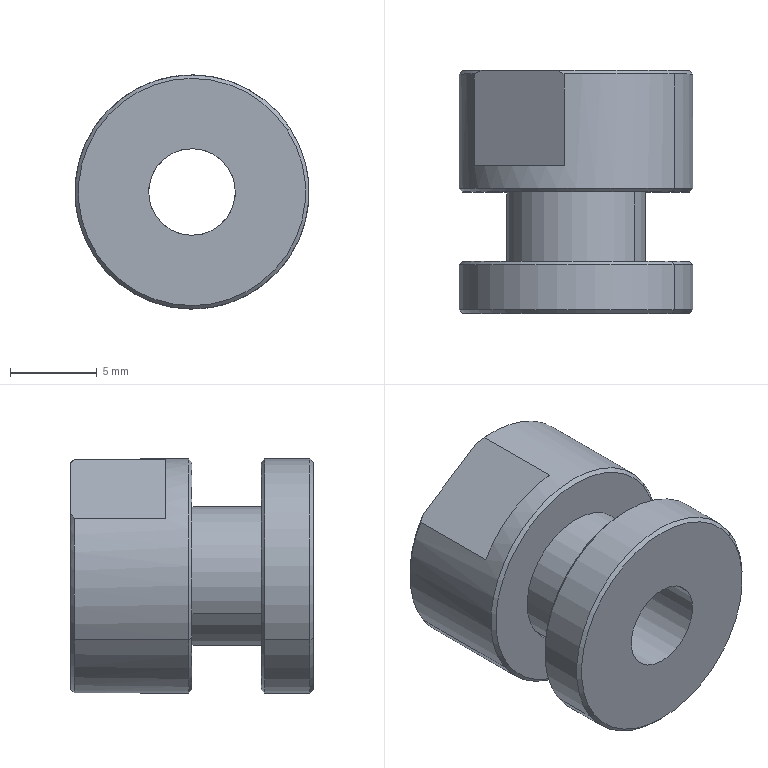Component | SolidWorks | WHC61-M5-0.8-L4.stp-1 | 1 solid | 25 faces | box 13.5 x 14 x 13.5 mm | volume 1320 mm3 | cone 9 | cylinder 8 | plane 8 | commonest cylinder face diameters 13.5 x4 5 x2 8 x2 | material AISI 304
STEP:
#1=COLOUR_RGB('',0.7922,0.8196,0.9333);
#2=FILL_AREA_STYLE_COLOUR('',#1);
#3=FILL_AREA_STYLE('',(#2));
#4=SURFACE_STYLE_FILL_AREA(#3);
#5=SURFACE_SIDE_STYLE('',(#4));
#6=SURFACE_STYLE_USAGE(.BOTH.,#5);
#7=PRESENTATION_STYLE_ASSIGNMENT((#6));
#8=CARTESIAN_POINT('',(0.08246,-2.402,0.05374));
#9=VERTEX_POINT('',#8);
#10=CARTESIAN_POINT('',(-0.08246,-2.402,-0.05374));
#11=VERTEX_POINT('',#10);
#12=CARTESIAN_POINT('',(0.,-2.402,0.));
#13=DIRECTION('',(0.,-1.,-0.));
#14=DIRECTION('',(-0.8378,0.,-0.546));
#15=AXIS2_PLACEMENT_3D('',#12,#13,#14);
#16=CIRCLE('',#15,0.09843);
#17=EDGE_CURVE('',#9,#11,#16,.T.);
#18=ORIENTED_EDGE('',*,*,#17,.F.);
#19=CARTESIAN_POINT('',(0.08246,-2.953,0.05374));
#20=VERTEX_POINT('',#19);
#21=CARTESIAN_POINT('',(0.08246,-2.402,0.05374));
#22=DIRECTION('',(0.,-1.,-0.));
#23=VECTOR('',#22,39.37);
#24=LINE('',#21,#23);
#25=EDGE_CURVE('',#9,#20,#24,.T.);
#26=ORIENTED_EDGE('',*,*,#25,.T.);
#27=CARTESIAN_POINT('',(-0.08246,-2.953,-0.05374));
#28=VERTEX_POINT('',#27);
#29=CARTESIAN_POINT('',(0.08246,-2.953,0.05374));
#30=CARTESIAN_POINT('',(0.07542,-2.953,0.06454));
#31=CARTESIAN_POINT('',(0.06624,-2.953,0.07393));
#32=CARTESIAN_POINT('',(0.04498,-2.953,0.08849));
#33=CARTESIAN_POINT('',(0.03291,-2.953,0.09365));
#34=CARTESIAN_POINT('',(0.007696,-2.953,0.09897));
#35=CARTESIAN_POINT('',(-0.005434,-2.953,0.09912));
#36=CARTESIAN_POINT('',(-0.03076,-2.953,0.09438));
#37=CARTESIAN_POINT('',(-0.04295,-2.953,0.08949));
#38=CARTESIAN_POINT('',(-0.06454,-2.953,0.07542));
#39=CARTESIAN_POINT('',(-0.07393,-2.953,0.06624));
#40=CARTESIAN_POINT('',(-0.08849,-2.953,0.04498));
#41=CARTESIAN_POINT('',(-0.09365,-2.953,0.03291));
#42=CARTESIAN_POINT('',(-0.09897,-2.953,0.007696));
#43=CARTESIAN_POINT('',(-0.09912,-2.953,-0.005434));
#44=CARTESIAN_POINT('',(-0.09438,-2.953,-0.03076));
#45=CARTESIAN_POINT('',(-0.08949,-2.953,-0.04295));
#46=CARTESIAN_POINT('',(-0.08246,-2.953,-0.05374));
#47=B_SPLINE_CURVE_WITH_KNOTS('',3,(#29,#30,#31,#32,#33,#34,#35,#36,#37,#38,#39,#40,#41,#42,#43,#44,#45,#46),.UNSPECIFIED.,.F.,.F.,(4,2,2,2,2,2,2,2,4),(0.5,0.5625,0.625,0.6875,0.75,0.8125,0.875,0.9375,1.),.UNSPECIFIED.);
#48=EDGE_CURVE('',#20,#28,#47,.T.);
#49=ORIENTED_EDGE('',*,*,#48,.T.);
#50=CARTESIAN_POINT('',(-0.08246,-2.402,-0.05374));
#51=DIRECTION('',(0.,-1.,-0.));
#52=VECTOR('',#51,39.37);
#53=LINE('',#50,#52);
#54=EDGE_CURVE('',#11,#28,#53,.T.);
#55=ORIENTED_EDGE('',*,*,#54,.F.);
#56=EDGE_LOOP('',(#18,#26,#49,#55));
#57=FACE_OUTER_BOUND('',#56,.T.);
#58=CARTESIAN_POINT('',(0.,-2.402,0.));
#59=DIRECTION('',(0.,-1.,-0.));
#60=DIRECTION('',(-0.8378,0.,-0.546));
#61=AXIS2_PLACEMENT_3D('',#58,#59,#60);
#62=CYLINDRICAL_SURFACE('',#61,0.09843);
#63=ADVANCED_FACE('',(#57),#62,.F.);
#64=CARTESIAN_POINT('',(-0.1319,-2.677,-0.08599));
#65=VERTEX_POINT('',#64);
#66=CARTESIAN_POINT('',(0.1319,-2.677,0.08599));
#67=VERTEX_POINT('',#66);
#68=CARTESIAN_POINT('',(0.,-2.677,0.));
#69=DIRECTION('',(-0.,1.,0.));
#70=DIRECTION('',(0.8378,0.,0.546));
#71=AXIS2_PLACEMENT_3D('',#68,#69,#70);
#72=CIRCLE('',#71,0.1575);
#73=EDGE_CURVE('',#65,#67,#72,.T.);
#74=ORIENTED_EDGE('',*,*,#73,.F.);
#75=CARTESIAN_POINT('',(-0.1319,-2.835,-0.08599));
#76=VERTEX_POINT('',#75);
#77=CARTESIAN_POINT('',(-0.1319,-0.9843,-0.08599));
#78=DIRECTION('',(0.,-1.,-0.));
#79=VECTOR('',#78,39.37);
#80=LINE('',#77,#79);
#81=EDGE_CURVE('',#65,#76,#80,.T.);
#82=ORIENTED_EDGE('',*,*,#81,.T.);
#83=CARTESIAN_POINT('',(0.1319,-2.835,0.08599));
#84=VERTEX_POINT('',#83);
#85=CARTESIAN_POINT('',(0.,-2.835,0.));
#86=DIRECTION('',(-0.,1.,0.));
#87=DIRECTION('',(0.8378,0.,0.546));
#88=AXIS2_PLACEMENT_3D('',#85,#86,#87);
#89=CIRCLE('',#88,0.1575);
#90=EDGE_CURVE('',#76,#84,#89,.T.);
#91=ORIENTED_EDGE('',*,*,#90,.T.);
#92=CARTESIAN_POINT('',(0.1319,-0.9843,0.08599));
#93=DIRECTION('',(0.,-1.,-0.));
#94=VECTOR('',#93,39.37);
#95=LINE('',#92,#94);
#96=EDGE_CURVE('',#67,#84,#95,.T.);
#97=ORIENTED_EDGE('',*,*,#96,.F.);
#98=EDGE_LOOP('',(#74,#82,#91,#97));
#99=FACE_OUTER_BOUND('',#98,.T.);
#100=CARTESIAN_POINT('',(-0.,-0.9843,0.));
#101=DIRECTION('',(0.,-1.,-0.));
#102=DIRECTION('',(0.8378,0.,0.546));
#103=AXIS2_PLACEMENT_3D('',#100,#101,#102);
#104=CYLINDRICAL_SURFACE('',#103,0.1575);
#105=ADVANCED_FACE('',(#99),#104,.T.);
#106=CARTESIAN_POINT('',(0.216,-2.835,0.1408));
#107=VERTEX_POINT('',#106);
#108=CARTESIAN_POINT('',(-0.216,-2.835,-0.1408));
#109=VERTEX_POINT('',#108);
#110=CARTESIAN_POINT('',(0.,-2.835,0.));
#111=DIRECTION('',(-0.,1.,0.));
#112=DIRECTION('',(0.8378,0.,0.546));
#113=AXIS2_PLACEMENT_3D('',#110,#111,#112);
#114=CIRCLE('',#113,0.2579);
#115=EDGE_CURVE('',#107,#109,#114,.T.);
#116=ORIENTED_EDGE('',*,*,#115,.F.);
#117=CARTESIAN_POINT('',(0.2226,-2.843,0.1451));
#118=VERTEX_POINT('',#117);
#119=CARTESIAN_POINT('',(0.2226,-2.843,0.1451));
#120=DIRECTION('',(0.5924,-0.7071,0.3861));
#121=VECTOR('',#120,39.37);
#122=LINE('',#119,#121);
#123=EDGE_CURVE('',#107,#118,#122,.T.);
#124=ORIENTED_EDGE('',*,*,#123,.T.);
#125=CARTESIAN_POINT('',(-0.2226,-2.843,-0.1451));
#126=VERTEX_POINT('',#125);
#127=CARTESIAN_POINT('',(0.,-2.843,0.));
#128=DIRECTION('',(-0.,1.,0.));
#129=DIRECTION('',(0.8378,0.,0.546));
#130=AXIS2_PLACEMENT_3D('',#127,#128,#129);
#131=CIRCLE('',#130,0.2657);
#132=EDGE_CURVE('',#118,#126,#131,.T.);
#133=ORIENTED_EDGE('',*,*,#132,.T.);
#134=CARTESIAN_POINT('',(-0.2226,-2.843,-0.1451));
#135=DIRECTION('',(-0.5924,-0.7071,-0.3861));
#136=VECTOR('',#135,39.37);
#137=LINE('',#134,#136);
#138=EDGE_CURVE('',#109,#126,#137,.T.);
#139=ORIENTED_EDGE('',*,*,#138,.F.);
#140=EDGE_LOOP('',(#116,#124,#133,#139));
#141=FACE_OUTER_BOUND('',#140,.T.);
#142=CARTESIAN_POINT('',(0.,-2.843,0.));
#143=DIRECTION('',(0.,-1.,-0.));
#144=DIRECTION('',(-0.8378,0.,-0.546));
#145=AXIS2_PLACEMENT_3D('',#142,#143,#144);
#146=CONICAL_SURFACE('',#145,0.2657,0.7854);
#147=ADVANCED_FACE('',(#141),#146,.T.);
#148=CARTESIAN_POINT('',(0.,-2.843,0.));
#149=DIRECTION('',(-0.,1.,0.));
#150=DIRECTION('',(0.8378,0.,0.546));
#151=AXIS2_PLACEMENT_3D('',#148,#149,#150);
#152=CIRCLE('',#151,0.2657);
#153=EDGE_CURVE('',#126,#118,#152,.T.);
#154=ORIENTED_EDGE('',*,*,#153,.F.);
#155=CARTESIAN_POINT('',(-0.2226,-2.945,-0.1451));
#156=VERTEX_POINT('',#155);
#157=CARTESIAN_POINT('',(-0.2226,-0.9843,-0.1451));
#158=DIRECTION('',(0.,-1.,-0.));
#159=VECTOR('',#158,39.37);
#160=LINE('',#157,#159);
#161=EDGE_CURVE('',#126,#156,#160,.T.);
#162=ORIENTED_EDGE('',*,*,#161,.T.);
#163=CARTESIAN_POINT('',(0.2226,-2.945,0.1451));
#164=VERTEX_POINT('',#163);
#165=CARTESIAN_POINT('',(0.,-2.945,0.));
#166=DIRECTION('',(-0.,1.,0.));
#167=DIRECTION('',(0.8378,0.,0.546));
#168=AXIS2_PLACEMENT_3D('',#165,#166,#167);
#169=CIRCLE('',#168,0.2657);
#170=EDGE_CURVE('',#156,#164,#169,.T.);
#171=ORIENTED_EDGE('',*,*,#170,.T.);
#172=CARTESIAN_POINT('',(0.2226,-0.9843,0.1451));
#173=DIRECTION('',(0.,-1.,-0.));
#174=VECTOR('',#173,39.37);
#175=LINE('',#172,#174);
#176=EDGE_CURVE('',#118,#164,#175,.T.);
#177=ORIENTED_EDGE('',*,*,#176,.F.);
#178=EDGE_LOOP('',(#154,#162,#171,#177));
#179=FACE_OUTER_BOUND('',#178,.T.);
#180=CARTESIAN_POINT('',(-0.,-0.9843,0.));
#181=DIRECTION('',(0.,-1.,-0.));
#182=DIRECTION('',(0.8378,0.,0.546));
#183=AXIS2_PLACEMENT_3D('',#180,#181,#182);
#184=CYLINDRICAL_SURFACE('',#183,0.2657);
#185=ADVANCED_FACE('',(#179),#184,.T.);
#186=CARTESIAN_POINT('',(0.216,-2.953,0.1408));
#187=VERTEX_POINT('',#186);
#188=CARTESIAN_POINT('',(-0.216,-2.953,-0.1408));
#189=VERTEX_POINT('',#188);
#190=CARTESIAN_POINT('',(0.,-2.953,0.));
#191=DIRECTION('',(-0.,1.,0.));
#192=DIRECTION('',(0.8378,0.,0.546));
#193=AXIS2_PLACEMENT_3D('',#190,#191,#192);
#194=CIRCLE('',#193,0.2579);
#195=EDGE_CURVE('',#187,#189,#194,.T.);
#196=ORIENTED_EDGE('',*,*,#195,.T.);
#197=CARTESIAN_POINT('',(-0.216,-2.953,-0.1408));
#198=DIRECTION('',(-0.5924,0.7071,-0.3861));
#199=VECTOR('',#198,39.37);
#200=LINE('',#197,#199);
#201=EDGE_CURVE('',#189,#156,#200,.T.);
#202=ORIENTED_EDGE('',*,*,#201,.T.);
#203=CARTESIAN_POINT('',(0.,-2.945,0.));
#204=DIRECTION('',(-0.,1.,0.));
#205=DIRECTION('',(0.8378,0.,0.546));
#206=AXIS2_PLACEMENT_3D('',#203,#204,#205);
#207=CIRCLE('',#206,0.2657);
#208=EDGE_CURVE('',#164,#156,#207,.T.);
#209=ORIENTED_EDGE('',*,*,#208,.F.);
#210=CARTESIAN_POINT('',(0.216,-2.953,0.1408));
#211=DIRECTION('',(0.5924,0.7071,0.3861));
#212=VECTOR('',#211,39.37);
#213=LINE('',#210,#212);
#214=EDGE_CURVE('',#187,#164,#213,.T.);
#215=ORIENTED_EDGE('',*,*,#214,.F.);
#216=EDGE_LOOP('',(#196,#202,#209,#215));
#217=FACE_OUTER_BOUND('',#216,.T.);
#218=CARTESIAN_POINT('',(0.,-2.953,0.));
#219=DIRECTION('',(-0.,1.,0.));
#220=DIRECTION('',(0.8378,0.,0.546));
#221=AXIS2_PLACEMENT_3D('',#218,#219,#220);
#222=CONICAL_SURFACE('',#221,0.2579,0.7854);
#223=ADVANCED_FACE('',(#217),#222,.T.);
#224=CARTESIAN_POINT('',(0.216,-2.677,0.1408));
#225=VERTEX_POINT('',#224);
#226=CARTESIAN_POINT('',(-0.216,-2.677,-0.1408));
#227=VERTEX_POINT('',#226);
#228=CARTESIAN_POINT('',(0.,-2.677,0.));
#229=DIRECTION('',(-0.,1.,0.));
#230=DIRECTION('',(0.8378,0.,0.546));
#231=AXIS2_PLACEMENT_3D('',#228,#229,#230);
#232=CIRCLE('',#231,0.2579);
#233=EDGE_CURVE('',#225,#227,#232,.T.);
#234=ORIENTED_EDGE('',*,*,#233,.T.);
#235=CARTESIAN_POINT('',(-0.2226,-2.669,-0.1451));
#236=VERTEX_POINT('',#235);
#237=CARTESIAN_POINT('',(-0.216,-2.677,-0.1408));
#238=DIRECTION('',(-0.5924,0.7071,-0.3861));
#239=VECTOR('',#238,39.37);
#240=LINE('',#237,#239);
#241=EDGE_CURVE('',#227,#236,#240,.T.);
#242=ORIENTED_EDGE('',*,*,#241,.T.);
#243=CARTESIAN_POINT('',(0.2226,-2.669,0.1451));
#244=VERTEX_POINT('',#243);
#245=CARTESIAN_POINT('',(0.,-2.669,0.));
#246=DIRECTION('',(-0.,1.,0.));
#247=DIRECTION('',(0.8378,0.,0.546));
#248=AXIS2_PLACEMENT_3D('',#245,#246,#247);
#249=CIRCLE('',#248,0.2657);
#250=EDGE_CURVE('',#244,#236,#249,.T.);
#251=ORIENTED_EDGE('',*,*,#250,.F.);
#252=CARTESIAN_POINT('',(0.216,-2.677,0.1408));
#253=DIRECTION('',(0.5924,0.7071,0.3861));
#254=VECTOR('',#253,39.37);
#255=LINE('',#252,#254);
#256=EDGE_CURVE('',#225,#244,#255,.T.);
#257=ORIENTED_EDGE('',*,*,#256,.F.);
#258=EDGE_LOOP('',(#234,#242,#251,#257));
#259=FACE_OUTER_BOUND('',#258,.T.);
#260=CARTESIAN_POINT('',(0.,-2.677,0.));
#261=DIRECTION('',(-0.,1.,0.));
#262=DIRECTION('',(0.8378,0.,0.546));
#263=AXIS2_PLACEMENT_3D('',#260,#261,#262);
#264=CONICAL_SURFACE('',#263,0.2579,0.7854);
#265=ADVANCED_FACE('',(#259),#264,.T.);
#266=CARTESIAN_POINT('',(-0.216,-2.402,-0.1408));
#267=VERTEX_POINT('',#266);
#268=CARTESIAN_POINT('',(-0.2156,-2.402,0.1414));
#269=VERTEX_POINT('',#268);
#270=CARTESIAN_POINT('',(0.,-2.402,0.));
#271=DIRECTION('',(-0.,1.,0.));
#272=DIRECTION('',(0.8378,0.,0.546));
#273=AXIS2_PLACEMENT_3D('',#270,#271,#272);
#274=CIRCLE('',#273,0.2579);
#275=EDGE_CURVE('',#267,#269,#274,.T.);
#276=ORIENTED_EDGE('',*,*,#275,.F.);
#277=CARTESIAN_POINT('',(-0.2226,-2.409,-0.1451));
#278=VERTEX_POINT('',#277);
#279=CARTESIAN_POINT('',(-0.2226,-2.409,-0.1451));
#280=DIRECTION('',(-0.5924,-0.7071,-0.3861));
#281=VECTOR('',#280,39.37);
#282=LINE('',#279,#281);
#283=EDGE_CURVE('',#267,#278,#282,.T.);
#284=ORIENTED_EDGE('',*,*,#283,.T.);
#285=CARTESIAN_POINT('',(-0.231,-2.409,0.1314));
#286=VERTEX_POINT('',#285);
#287=CARTESIAN_POINT('',(0.,-2.409,0.));
#288=DIRECTION('',(-0.,1.,0.));
#289=DIRECTION('',(0.8378,0.,0.546));
#290=AXIS2_PLACEMENT_3D('',#287,#288,#289);
#291=CIRCLE('',#290,0.2657);
#292=EDGE_CURVE('',#278,#286,#291,.T.);
#293=ORIENTED_EDGE('',*,*,#292,.T.);
#294=CARTESIAN_POINT('',(-0.231,-2.409,0.1314));
#295=CARTESIAN_POINT('',(-0.2259,-2.407,0.1347));
#296=CARTESIAN_POINT('',(-0.2208,-2.404,0.138));
#297=CARTESIAN_POINT('',(-0.2156,-2.402,0.1414));
#298=B_SPLINE_CURVE_WITH_KNOTS('',3,(#294,#295,#296,#297),.UNSPECIFIED.,.F.,.F.,(4,4),(0.004377,0.00488),.UNSPECIFIED.);
#299=EDGE_CURVE('',#286,#269,#298,.T.);
#300=ORIENTED_EDGE('',*,*,#299,.T.);
#301=EDGE_LOOP('',(#276,#284,#293,#300));
#302=FACE_OUTER_BOUND('',#301,.T.);
#303=CARTESIAN_POINT('',(0.,-2.409,0.));
#304=DIRECTION('',(0.,-1.,-0.));
#305=DIRECTION('',(-0.8378,0.,-0.546));
#306=AXIS2_PLACEMENT_3D('',#303,#304,#305);
#307=CONICAL_SURFACE('',#306,0.2657,0.7854);
#308=ADVANCED_FACE('',(#302),#307,.T.);
#309=ORIENTED_EDGE('',*,*,#292,.F.);
#310=CARTESIAN_POINT('',(-0.2226,-0.9843,-0.1451));
#311=DIRECTION('',(0.,-1.,-0.));
#312=VECTOR('',#311,39.37);
#313=LINE('',#310,#312);
#314=EDGE_CURVE('',#278,#236,#313,.T.);
#315=ORIENTED_EDGE('',*,*,#314,.T.);
#316=CARTESIAN_POINT('',(0.,-2.669,0.));
#317=DIRECTION('',(-0.,1.,0.));
#318=DIRECTION('',(0.8378,0.,0.546));
#319=AXIS2_PLACEMENT_3D('',#316,#317,#318);
#320=CIRCLE('',#319,0.2657);
#321=EDGE_CURVE('',#236,#244,#320,.T.);
#322=ORIENTED_EDGE('',*,*,#321,.T.);
#323=CARTESIAN_POINT('',(0.2226,-2.409,0.1451));
#324=VERTEX_POINT('',#323);
#325=CARTESIAN_POINT('',(0.2226,-0.9843,0.1451));
#326=DIRECTION('',(0.,-1.,-0.));
#327=VECTOR('',#326,39.37);
#328=LINE('',#325,#327);
#329=EDGE_CURVE('',#324,#244,#328,.T.);
#330=ORIENTED_EDGE('',*,*,#329,.F.);
#331=CARTESIAN_POINT('',(-0.02699,-2.409,0.2644));
#332=VERTEX_POINT('',#331);
#333=CARTESIAN_POINT('',(0.,-2.409,0.));
#334=DIRECTION('',(-0.,1.,0.));
#335=DIRECTION('',(0.8378,0.,0.546));
#336=AXIS2_PLACEMENT_3D('',#333,#334,#335);
#337=CIRCLE('',#336,0.2657);
#338=EDGE_CURVE('',#332,#324,#337,.T.);
#339=ORIENTED_EDGE('',*,*,#338,.F.);
#340=CARTESIAN_POINT('',(-0.02699,-2.618,0.2644));
#341=VERTEX_POINT('',#340);
#342=CARTESIAN_POINT('',(-0.02699,-2.618,0.2644));
#343=DIRECTION('',(-0.,1.,0.));
#344=VECTOR('',#343,39.37);
#345=LINE('',#342,#344);
#346=EDGE_CURVE('',#341,#332,#345,.T.);
#347=ORIENTED_EDGE('',*,*,#346,.F.);
#348=CARTESIAN_POINT('',(-0.231,-2.618,0.1314));
#349=VERTEX_POINT('',#348);
#350=CARTESIAN_POINT('',(0.,-2.618,0.));
#351=DIRECTION('',(-0.,1.,0.));
#352=DIRECTION('',(0.546,0.,-0.8378));
#353=AXIS2_PLACEMENT_3D('',#350,#351,#352);
#354=CIRCLE('',#353,0.2657);
#355=EDGE_CURVE('',#349,#341,#354,.T.);
#356=ORIENTED_EDGE('',*,*,#355,.F.);
#357=CARTESIAN_POINT('',(-0.231,-2.618,0.1314));
#358=DIRECTION('',(-0.,1.,0.));
#359=VECTOR('',#358,39.37);
#360=LINE('',#357,#359);
#361=EDGE_CURVE('',#349,#286,#360,.T.);
#362=ORIENTED_EDGE('',*,*,#361,.T.);
#363=EDGE_LOOP('',(#309,#315,#322,#330,#339,#347,#356,#362));
#364=FACE_OUTER_BOUND('',#363,.T.);
#365=CARTESIAN_POINT('',(-0.,-0.9843,0.));
#366=DIRECTION('',(0.,-1.,-0.));
#367=DIRECTION('',(0.8378,0.,0.546));
#368=AXIS2_PLACEMENT_3D('',#365,#366,#367);
#369=CYLINDRICAL_SURFACE('',#368,0.2657);
#370=ADVANCED_FACE('',(#364),#369,.T.);
#371=ORIENTED_EDGE('',*,*,#195,.F.);
#372=CARTESIAN_POINT('',(0.,-2.953,0.));
#373=DIRECTION('',(-0.,1.,0.));
#374=DIRECTION('',(0.8378,0.,0.546));
#375=AXIS2_PLACEMENT_3D('',#372,#373,#374);
#376=CIRCLE('',#375,0.2579);
#377=EDGE_CURVE('',#189,#187,#376,.T.);
#378=ORIENTED_EDGE('',*,*,#377,.F.);
#379=EDGE_LOOP('',(#371,#378));
#380=FACE_OUTER_BOUND('',#379,.T.);
#381=CARTESIAN_POINT('',(-0.08246,-2.953,-0.05374));
#382=CARTESIAN_POINT('',(-0.07542,-2.953,-0.06454));
#383=CARTESIAN_POINT('',(-0.06624,-2.953,-0.07393));
#384=CARTESIAN_POINT('',(-0.04498,-2.953,-0.08849));
#385=CARTESIAN_POINT('',(-0.03291,-2.953,-0.09365));
#386=CARTESIAN_POINT('',(-0.007696,-2.953,-0.09897));
#387=CARTESIAN_POINT('',(0.005434,-2.953,-0.09912));
#388=CARTESIAN_POINT('',(0.03076,-2.953,-0.09438));
#389=CARTESIAN_POINT('',(0.04295,-2.953,-0.08949));
#390=CARTESIAN_POINT('',(0.06454,-2.953,-0.07542));
#391=CARTESIAN_POINT('',(0.07393,-2.953,-0.06624));
#392=CARTESIAN_POINT('',(0.08849,-2.953,-0.04498));
#393=CARTESIAN_POINT('',(0.09365,-2.953,-0.03291));
#394=CARTESIAN_POINT('',(0.09897,-2.953,-0.007696));
#395=CARTESIAN_POINT('',(0.09912,-2.953,0.005434));
#396=CARTESIAN_POINT('',(0.09438,-2.953,0.03076));
#397=CARTESIAN_POINT('',(0.08949,-2.953,0.04295));
#398=CARTESIAN_POINT('',(0.08246,-2.953,0.05374));
#399=B_SPLINE_CURVE_WITH_KNOTS('',3,(#381,#382,#383,#384,#385,#386,#387,#388,#389,#390,#391,#392,#393,#394,#395,#396,#397,#398),.UNSPECIFIED.,.F.,.F.,(4,2,2,2,2,2,2,2,4),(0.,0.0625,0.125,0.1875,0.25,0.3125,0.375,0.4375,0.5),.UNSPECIFIED.);
#400=EDGE_CURVE('',#28,#20,#399,.T.);
#401=ORIENTED_EDGE('',*,*,#400,.F.);
#402=ORIENTED_EDGE('',*,*,#48,.F.);
#403=EDGE_LOOP('',(#401,#402));
#404=FACE_BOUND('',#403,.T.);
#405=CARTESIAN_POINT('',(0.,-2.953,0.));
#406=DIRECTION('',(-0.,1.,0.));
#407=DIRECTION('',(-0.546,-0.,0.8378));
#408=AXIS2_PLACEMENT_3D('',#405,#406,#407);
#409=PLANE('',#408);
#410=ADVANCED_FACE('',(#380,#404),#409,.F.);
#411=ORIENTED_EDGE('',*,*,#361,.F.);
#412=CARTESIAN_POINT('',(-0.02699,-2.618,0.2644));
#413=DIRECTION('',(-0.8378,-0.,-0.546));
#414=VECTOR('',#413,39.37);
#415=LINE('',#412,#414);
#416=EDGE_CURVE('',#341,#349,#415,.T.);
#417=ORIENTED_EDGE('',*,*,#416,.F.);
#418=ORIENTED_EDGE('',*,*,#346,.T.);
#419=CARTESIAN_POINT('',(-0.04233,-2.402,0.2544));
#420=VERTEX_POINT('',#419);
#421=CARTESIAN_POINT('',(-0.04233,-2.402,0.2544));
#422=CARTESIAN_POINT('',(-0.03717,-2.404,0.2577));
#423=CARTESIAN_POINT('',(-0.03205,-2.407,0.2611));
#424=CARTESIAN_POINT('',(-0.02699,-2.409,0.2644));
#425=B_SPLINE_CURVE_WITH_KNOTS('',3,(#421,#422,#423,#424),.UNSPECIFIED.,.F.,.F.,(4,4),(0.01023,0.01072),.UNSPECIFIED.);
#426=EDGE_CURVE('',#420,#332,#425,.T.);
#427=ORIENTED_EDGE('',*,*,#426,.F.);
#428=CARTESIAN_POINT('',(-0.129,-2.402,0.1979));
#429=DIRECTION('',(0.8378,0.,0.546));
#430=VECTOR('',#429,39.37);
#431=LINE('',#428,#430);
#432=EDGE_CURVE('',#269,#420,#431,.T.);
#433=ORIENTED_EDGE('',*,*,#432,.F.);
#434=ORIENTED_EDGE('',*,*,#299,.F.);
#435=EDGE_LOOP('',(#411,#417,#418,#427,#433,#434));
#436=FACE_OUTER_BOUND('',#435,.T.);
#437=CARTESIAN_POINT('',(-0.02699,-2.618,0.2644));
#438=DIRECTION('',(0.546,0.,-0.8378));
#439=DIRECTION('',(-0.8378,-0.,-0.546));
#440=AXIS2_PLACEMENT_3D('',#437,#438,#439);
#441=PLANE('',#440);
#442=ADVANCED_FACE('',(#436),#441,.F.);
#443=ORIENTED_EDGE('',*,*,#416,.T.);
#444=ORIENTED_EDGE('',*,*,#355,.T.);
#445=EDGE_LOOP('',(#443,#444));
#446=FACE_OUTER_BOUND('',#445,.T.);
#447=CARTESIAN_POINT('',(0.,-2.618,0.));
#448=DIRECTION('',(-0.,1.,0.));
#449=DIRECTION('',(-0.546,-0.,0.8378));
#450=AXIS2_PLACEMENT_3D('',#447,#448,#449);
#451=PLANE('',#450);
#452=ADVANCED_FACE('',(#446),#451,.T.);
#453=ORIENTED_EDGE('',*,*,#314,.F.);
#454=CARTESIAN_POINT('',(0.02699,-2.409,-0.2644));
#455=VERTEX_POINT('',#454);
#456=CARTESIAN_POINT('',(0.,-2.409,0.));
#457=DIRECTION('',(-0.,1.,0.));
#458=DIRECTION('',(0.8378,0.,0.546));
#459=AXIS2_PLACEMENT_3D('',#456,#457,#458);
#460=CIRCLE('',#459,0.2657);
#461=EDGE_CURVE('',#455,#278,#460,.T.);
#462=ORIENTED_EDGE('',*,*,#461,.F.);
#463=CARTESIAN_POINT('',(0.02699,-2.618,-0.2644));
#464=VERTEX_POINT('',#463);
#465=CARTESIAN_POINT('',(0.02699,-2.618,-0.2644));
#466=DIRECTION('',(-0.,1.,0.));
#467=VECTOR('',#466,39.37);
#468=LINE('',#465,#467);
#469=EDGE_CURVE('',#464,#455,#468,.T.);
#470=ORIENTED_EDGE('',*,*,#469,.F.);
#471=CARTESIAN_POINT('',(0.231,-2.618,-0.1314));
#472=VERTEX_POINT('',#471);
#473=CARTESIAN_POINT('',(0.,-2.618,0.));
#474=DIRECTION('',(-0.,1.,0.));
#475=DIRECTION('',(0.546,0.,-0.8378));
#476=AXIS2_PLACEMENT_3D('',#473,#474,#475);
#477=CIRCLE('',#476,0.2657);
#478=EDGE_CURVE('',#472,#464,#477,.T.);
#479=ORIENTED_EDGE('',*,*,#478,.F.);
#480=CARTESIAN_POINT('',(0.231,-2.409,-0.1314));
#481=VERTEX_POINT('',#480);
#482=CARTESIAN_POINT('',(0.231,-2.618,-0.1314));
#483=DIRECTION('',(-0.,1.,0.));
#484=VECTOR('',#483,39.37);
#485=LINE('',#482,#484);
#486=EDGE_CURVE('',#472,#481,#485,.T.);
#487=ORIENTED_EDGE('',*,*,#486,.T.);
#488=CARTESIAN_POINT('',(0.,-2.409,0.));
#489=DIRECTION('',(-0.,1.,0.));
#490=DIRECTION('',(0.8378,0.,0.546));
#491=AXIS2_PLACEMENT_3D('',#488,#489,#490);
#492=CIRCLE('',#491,0.2657);
#493=EDGE_CURVE('',#324,#481,#492,.T.);
#494=ORIENTED_EDGE('',*,*,#493,.F.);
#495=ORIENTED_EDGE('',*,*,#329,.T.);
#496=ORIENTED_EDGE('',*,*,#250,.T.);
#497=EDGE_LOOP('',(#453,#462,#470,#479,#487,#494,#495,#496));
#498=FACE_OUTER_BOUND('',#497,.T.);
#499=CARTESIAN_POINT('',(-0.,-0.9843,0.));
#500=DIRECTION('',(0.,-1.,-0.));
#501=DIRECTION('',(0.8378,0.,0.546));
#502=AXIS2_PLACEMENT_3D('',#499,#500,#501);
#503=CYLINDRICAL_SURFACE('',#502,0.2657);
#504=ADVANCED_FACE('',(#498),#503,.T.);
#505=CARTESIAN_POINT('',(0.2156,-2.402,-0.1414));
#506=VERTEX_POINT('',#505);
#507=CARTESIAN_POINT('',(0.,-2.402,0.));
#508=DIRECTION('',(-0.,1.,0.));
#509=DIRECTION('',(0.8378,0.,0.546));
#510=AXIS2_PLACEMENT_3D('',#507,#508,#509);
#511=CIRCLE('',#510,0.2579);
#512=EDGE_CURVE('',#420,#506,#511,.T.);
#513=ORIENTED_EDGE('',*,*,#512,.F.);
#514=ORIENTED_EDGE('',*,*,#426,.T.);
#515=ORIENTED_EDGE('',*,*,#338,.T.);
#516=ORIENTED_EDGE('',*,*,#493,.T.);
#517=CARTESIAN_POINT('',(0.231,-2.409,-0.1314));
#518=CARTESIAN_POINT('',(0.2259,-2.407,-0.1347));
#519=CARTESIAN_POINT('',(0.2208,-2.404,-0.138));
#520=CARTESIAN_POINT('',(0.2156,-2.402,-0.1414));
#521=B_SPLINE_CURVE_WITH_KNOTS('',3,(#517,#518,#519,#520),.UNSPECIFIED.,.F.,.F.,(4,4),(0.004377,0.00488),.UNSPECIFIED.);
#522=EDGE_CURVE('',#481,#506,#521,.T.);
#523=ORIENTED_EDGE('',*,*,#522,.T.);
#524=EDGE_LOOP('',(#513,#514,#515,#516,#523));
#525=FACE_OUTER_BOUND('',#524,.T.);
#526=CARTESIAN_POINT('',(0.,-2.409,0.));
#527=DIRECTION('',(0.,-1.,-0.));
#528=DIRECTION('',(-0.8378,0.,-0.546));
#529=AXIS2_PLACEMENT_3D('',#526,#527,#528);
#530=CONICAL_SURFACE('',#529,0.2657,0.7854);
#531=ADVANCED_FACE('',(#525),#530,.T.);
#532=CARTESIAN_POINT('',(0.02699,-2.618,-0.2644));
#533=DIRECTION('',(0.8378,0.,0.546));
#534=VECTOR('',#533,39.37);
#535=LINE('',#532,#534);
#536=EDGE_CURVE('',#464,#472,#535,.T.);
#537=ORIENTED_EDGE('',*,*,#536,.T.);
#538=ORIENTED_EDGE('',*,*,#478,.T.);
#539=EDGE_LOOP('',(#537,#538));
#540=FACE_OUTER_BOUND('',#539,.T.);
#541=CARTESIAN_POINT('',(0.,-2.618,0.));
#542=DIRECTION('',(-0.,1.,0.));
#543=DIRECTION('',(-0.546,-0.,0.8378));
#544=AXIS2_PLACEMENT_3D('',#541,#542,#543);
#545=PLANE('',#544);
#546=ADVANCED_FACE('',(#540),#545,.T.);
#547=ORIENTED_EDGE('',*,*,#486,.F.);
#548=ORIENTED_EDGE('',*,*,#536,.F.);
#549=ORIENTED_EDGE('',*,*,#469,.T.);
#550=CARTESIAN_POINT('',(0.04233,-2.402,-0.2544));
#551=VERTEX_POINT('',#550);
#552=CARTESIAN_POINT('',(0.04233,-2.402,-0.2544));
#553=CARTESIAN_POINT('',(0.03717,-2.404,-0.2577));
#554=CARTESIAN_POINT('',(0.03205,-2.407,-0.2611));
#555=CARTESIAN_POINT('',(0.02699,-2.409,-0.2644));
#556=B_SPLINE_CURVE_WITH_KNOTS('',3,(#552,#553,#554,#555),.UNSPECIFIED.,.F.,.F.,(4,4),(0.01023,0.01072),.UNSPECIFIED.);
#557=EDGE_CURVE('',#551,#455,#556,.T.);
#558=ORIENTED_EDGE('',*,*,#557,.F.);
#559=CARTESIAN_POINT('',(0.129,-2.402,-0.1979));
#560=DIRECTION('',(-0.8378,-0.,-0.546));
#561=VECTOR('',#560,39.37);
#562=LINE('',#559,#561);
#563=EDGE_CURVE('',#506,#551,#562,.T.);
#564=ORIENTED_EDGE('',*,*,#563,.F.);
#565=ORIENTED_EDGE('',*,*,#522,.F.);
#566=EDGE_LOOP('',(#547,#548,#549,#558,#564,#565));
#567=FACE_OUTER_BOUND('',#566,.T.);
#568=CARTESIAN_POINT('',(0.02699,-2.618,-0.2644));
#569=DIRECTION('',(-0.546,-0.,0.8378));
#570=DIRECTION('',(-0.,1.,0.));
#571=AXIS2_PLACEMENT_3D('',#568,#569,#570);
#572=PLANE('',#571);
#573=ADVANCED_FACE('',(#567),#572,.F.);
#574=ORIENTED_EDGE('',*,*,#512,.T.);
#575=ORIENTED_EDGE('',*,*,#563,.T.);
#576=CARTESIAN_POINT('',(0.,-2.402,0.));
#577=DIRECTION('',(-0.,1.,0.));
#578=DIRECTION('',(0.8378,0.,0.546));
#579=AXIS2_PLACEMENT_3D('',#576,#577,#578);
#580=CIRCLE('',#579,0.2579);
#581=EDGE_CURVE('',#551,#267,#580,.T.);
#582=ORIENTED_EDGE('',*,*,#581,.T.);
#583=ORIENTED_EDGE('',*,*,#275,.T.);
#584=ORIENTED_EDGE('',*,*,#432,.T.);
#585=EDGE_LOOP('',(#574,#575,#582,#583,#584));
#586=FACE_OUTER_BOUND('',#585,.T.);
#587=CARTESIAN_POINT('',(0.,-2.402,0.));
#588=DIRECTION('',(0.,-1.,-0.));
#589=DIRECTION('',(-0.8378,0.,-0.546));
#590=AXIS2_PLACEMENT_3D('',#587,#588,#589);
#591=CIRCLE('',#590,0.09843);
#592=EDGE_CURVE('',#11,#9,#591,.T.);
#593=ORIENTED_EDGE('',*,*,#592,.T.);
#594=ORIENTED_EDGE('',*,*,#17,.T.);
#595=EDGE_LOOP('',(#593,#594));
#596=FACE_BOUND('',#595,.T.);
#597=CARTESIAN_POINT('',(0.1408,-2.402,-0.216));
#598=DIRECTION('',(0.,-1.,-0.));
#599=DIRECTION('',(-0.8378,-0.,-0.546));
#600=AXIS2_PLACEMENT_3D('',#597,#598,#599);
#601=PLANE('',#600);
#602=ADVANCED_FACE('',(#586,#596),#601,.F.);
#603=ORIENTED_EDGE('',*,*,#283,.F.);
#604=ORIENTED_EDGE('',*,*,#581,.F.);
#605=ORIENTED_EDGE('',*,*,#557,.T.);
#606=ORIENTED_EDGE('',*,*,#461,.T.);
#607=EDGE_LOOP('',(#603,#604,#605,#606));
#608=FACE_OUTER_BOUND('',#607,.T.);
#609=CARTESIAN_POINT('',(0.,-2.409,0.));
#610=DIRECTION('',(0.,-1.,-0.));
#611=DIRECTION('',(-0.8378,0.,-0.546));
#612=AXIS2_PLACEMENT_3D('',#609,#610,#611);
#613=CONICAL_SURFACE('',#612,0.2657,0.7854);
#614=ADVANCED_FACE('',(#608),#613,.T.);
#615=ORIENTED_EDGE('',*,*,#241,.F.);
#616=CARTESIAN_POINT('',(0.,-2.677,0.));
#617=DIRECTION('',(-0.,1.,0.));
#618=DIRECTION('',(0.8378,0.,0.546));
#619=AXIS2_PLACEMENT_3D('',#616,#617,#618);
#620=CIRCLE('',#619,0.2579);
#621=EDGE_CURVE('',#227,#225,#620,.T.);
#622=ORIENTED_EDGE('',*,*,#621,.T.);
#623=ORIENTED_EDGE('',*,*,#256,.T.);
#624=ORIENTED_EDGE('',*,*,#321,.F.);
#625=EDGE_LOOP('',(#615,#622,#623,#624));
#626=FACE_OUTER_BOUND('',#625,.T.);
#627=CARTESIAN_POINT('',(0.,-2.677,0.));
#628=DIRECTION('',(-0.,1.,0.));
#629=DIRECTION('',(0.8378,0.,0.546));
#630=AXIS2_PLACEMENT_3D('',#627,#628,#629);
#631=CONICAL_SURFACE('',#630,0.2579,0.7854);
#632=ADVANCED_FACE('',(#626),#631,.T.);
#633=ORIENTED_EDGE('',*,*,#201,.F.);
#634=ORIENTED_EDGE('',*,*,#377,.T.);
#635=ORIENTED_EDGE('',*,*,#214,.T.);
#636=ORIENTED_EDGE('',*,*,#170,.F.);
#637=EDGE_LOOP('',(#633,#634,#635,#636));
#638=FACE_OUTER_BOUND('',#637,.T.);
#639=CARTESIAN_POINT('',(0.,-2.953,0.));
#640=DIRECTION('',(-0.,1.,0.));
#641=DIRECTION('',(0.8378,0.,0.546));
#642=AXIS2_PLACEMENT_3D('',#639,#640,#641);
#643=CONICAL_SURFACE('',#642,0.2579,0.7854);
#644=ADVANCED_FACE('',(#638),#643,.T.);
#645=ORIENTED_EDGE('',*,*,#161,.F.);
#646=ORIENTED_EDGE('',*,*,#132,.F.);
#647=ORIENTED_EDGE('',*,*,#176,.T.);
#648=ORIENTED_EDGE('',*,*,#208,.T.);
#649=EDGE_LOOP('',(#645,#646,#647,#648));
#650=FACE_OUTER_BOUND('',#649,.T.);
#651=CARTESIAN_POINT('',(-0.,-0.9843,0.));
#652=DIRECTION('',(0.,-1.,-0.));
#653=DIRECTION('',(0.8378,0.,0.546));
#654=AXIS2_PLACEMENT_3D('',#651,#652,#653);
#655=CYLINDRICAL_SURFACE('',#654,0.2657);
#656=ADVANCED_FACE('',(#650),#655,.T.);
#657=ORIENTED_EDGE('',*,*,#123,.F.);
#658=CARTESIAN_POINT('',(0.,-2.835,0.));
#659=DIRECTION('',(-0.,1.,0.));
#660=DIRECTION('',(0.8378,0.,0.546));
#661=AXIS2_PLACEMENT_3D('',#658,#659,#660);
#662=CIRCLE('',#661,0.2579);
#663=EDGE_CURVE('',#109,#107,#662,.T.);
#664=ORIENTED_EDGE('',*,*,#663,.F.);
#665=ORIENTED_EDGE('',*,*,#138,.T.);
#666=ORIENTED_EDGE('',*,*,#153,.T.);
#667=EDGE_LOOP('',(#657,#664,#665,#666));
#668=FACE_OUTER_BOUND('',#667,.T.);
#669=CARTESIAN_POINT('',(0.,-2.843,0.));
#670=DIRECTION('',(0.,-1.,-0.));
#671=DIRECTION('',(-0.8378,0.,-0.546));
#672=AXIS2_PLACEMENT_3D('',#669,#670,#671);
#673=CONICAL_SURFACE('',#672,0.2657,0.7854);
#674=ADVANCED_FACE('',(#668),#673,.T.);
#675=ORIENTED_EDGE('',*,*,#663,.T.);
#676=ORIENTED_EDGE('',*,*,#115,.T.);
#677=EDGE_LOOP('',(#675,#676));
#678=FACE_OUTER_BOUND('',#677,.T.);
#679=CARTESIAN_POINT('',(0.,-2.835,0.));
#680=DIRECTION('',(-0.,1.,0.));
#681=DIRECTION('',(0.8378,0.,0.546));
#682=AXIS2_PLACEMENT_3D('',#679,#680,#681);
#683=CIRCLE('',#682,0.1575);
#684=EDGE_CURVE('',#84,#76,#683,.T.);
#685=ORIENTED_EDGE('',*,*,#684,.F.);
#686=ORIENTED_EDGE('',*,*,#90,.F.);
#687=EDGE_LOOP('',(#685,#686));
#688=FACE_BOUND('',#687,.T.);
#689=CARTESIAN_POINT('',(0.1408,-2.835,-0.216));
#690=DIRECTION('',(0.,-1.,-0.));
#691=DIRECTION('',(-0.8378,-0.,-0.546));
#692=AXIS2_PLACEMENT_3D('',#689,#690,#691);
#693=PLANE('',#692);
#694=ADVANCED_FACE('',(#678,#688),#693,.F.);
#695=ORIENTED_EDGE('',*,*,#81,.F.);
#696=CARTESIAN_POINT('',(0.,-2.677,0.));
#697=DIRECTION('',(-0.,1.,0.));
#698=DIRECTION('',(0.8378,0.,0.546));
#699=AXIS2_PLACEMENT_3D('',#696,#697,#698);
#700=CIRCLE('',#699,0.1575);
#701=EDGE_CURVE('',#67,#65,#700,.T.);
#702=ORIENTED_EDGE('',*,*,#701,.F.);
#703=ORIENTED_EDGE('',*,*,#96,.T.);
#704=ORIENTED_EDGE('',*,*,#684,.T.);
#705=EDGE_LOOP('',(#695,#702,#703,#704));
#706=FACE_OUTER_BOUND('',#705,.T.);
#707=CARTESIAN_POINT('',(-0.,-0.9843,0.));
#708=DIRECTION('',(0.,-1.,-0.));
#709=DIRECTION('',(0.8378,0.,0.546));
#710=AXIS2_PLACEMENT_3D('',#707,#708,#709);
#711=CYLINDRICAL_SURFACE('',#710,0.1575);
#712=ADVANCED_FACE('',(#706),#711,.T.);
#713=ORIENTED_EDGE('',*,*,#233,.F.);
#714=ORIENTED_EDGE('',*,*,#621,.F.);
#715=EDGE_LOOP('',(#713,#714));
#716=FACE_OUTER_BOUND('',#715,.T.);
#717=ORIENTED_EDGE('',*,*,#701,.T.);
#718=ORIENTED_EDGE('',*,*,#73,.T.);
#719=EDGE_LOOP('',(#717,#718));
#720=FACE_BOUND('',#719,.T.);
#721=CARTESIAN_POINT('',(0.08599,-2.677,-0.1319));
#722=DIRECTION('',(-0.,1.,0.));
#723=DIRECTION('',(-0.546,-0.,0.8378));
#724=AXIS2_PLACEMENT_3D('',#721,#722,#723);
#725=PLANE('',#724);
#726=ADVANCED_FACE('',(#716,#720),#725,.F.);
#727=ORIENTED_EDGE('',*,*,#25,.F.);
#728=ORIENTED_EDGE('',*,*,#592,.F.);
#729=ORIENTED_EDGE('',*,*,#54,.T.);
#730=ORIENTED_EDGE('',*,*,#400,.T.);
#731=EDGE_LOOP('',(#727,#728,#729,#730));
#732=FACE_OUTER_BOUND('',#731,.T.);
#733=CARTESIAN_POINT('',(0.,-2.402,0.));
#734=DIRECTION('',(0.,-1.,-0.));
#735=DIRECTION('',(-0.8378,0.,-0.546));
#736=AXIS2_PLACEMENT_3D('',#733,#734,#735);
#737=CYLINDRICAL_SURFACE('',#736,0.09843);
#738=ADVANCED_FACE('',(#732),#737,.F.);
#739=CLOSED_SHELL('',(#63,#105,#147,#185,#223,#265,#308,#370,#410,#442,#452,#504,#531,#546,#573,#602,#614,#632,#644,#656,#674,#694,#712,#726,#738));
#740=MANIFOLD_SOLID_BREP('',#739);
#741=STYLED_ITEM('',(#7),#740);
#742=PRESENTATION_LAYER_ASSIGNMENT('','',(#741));
#743=CARTESIAN_POINT('',(0.,0.,0.));
#744=DIRECTION('',(0.,0.,1.));
#745=DIRECTION('',(1.,0.,0.));
#746=AXIS2_PLACEMENT_3D('',#743,#744,#745);
#747=(LENGTH_UNIT()NAMED_UNIT(*)SI_UNIT($,.METRE.));
#748=LENGTH_MEASURE_WITH_UNIT(LENGTH_MEASURE(0.0254),#747);
#749=DIMENSIONAL_EXPONENTS(1.,0.,0.,0.,0.,0.,0.);
#750=(CONVERSION_BASED_UNIT('',#748)LENGTH_UNIT()NAMED_UNIT(#749));
#751=UNCERTAINTY_MEASURE_WITH_UNIT(LENGTH_MEASURE(0.00001),#750,'','');
#752=(NAMED_UNIT(*)PLANE_ANGLE_UNIT()SI_UNIT($,.RADIAN.));
#753=(NAMED_UNIT(*)SI_UNIT($,.STERADIAN.)SOLID_ANGLE_UNIT());
#754=(GEOMETRIC_REPRESENTATION_CONTEXT(3)GLOBAL_UNCERTAINTY_ASSIGNED_CONTEXT((#751))GLOBAL_UNIT_ASSIGNED_CONTEXT((#750,#752,#753))REPRESENTATION_CONTEXT('',''));
#755=ADVANCED_BREP_SHAPE_REPRESENTATION('',(#740,#746),#754);
#756=(LENGTH_UNIT()NAMED_UNIT(*)SI_UNIT($,.METRE.));
#757=LENGTH_MEASURE_WITH_UNIT(LENGTH_MEASURE(0.0254),#756);
#758=DIMENSIONAL_EXPONENTS(1.,0.,0.,0.,0.,0.,0.);
#759=(CONVERSION_BASED_UNIT('',#757)LENGTH_UNIT()NAMED_UNIT(#758));
#760=UNCERTAINTY_MEASURE_WITH_UNIT(LENGTH_MEASURE(0.00001),#759,'','');
#761=(NAMED_UNIT(*)PLANE_ANGLE_UNIT()SI_UNIT($,.RADIAN.));
#762=(NAMED_UNIT(*)SI_UNIT($,.STERADIAN.)SOLID_ANGLE_UNIT());
#763=(GEOMETRIC_REPRESENTATION_CONTEXT(3)GLOBAL_UNCERTAINTY_ASSIGNED_CONTEXT((#760))GLOBAL_UNIT_ASSIGNED_CONTEXT((#759,#761,#762))REPRESENTATION_CONTEXT('',''));
#764=MECHANICAL_DESIGN_GEOMETRIC_PRESENTATION_REPRESENTATION('',(#741),#763);